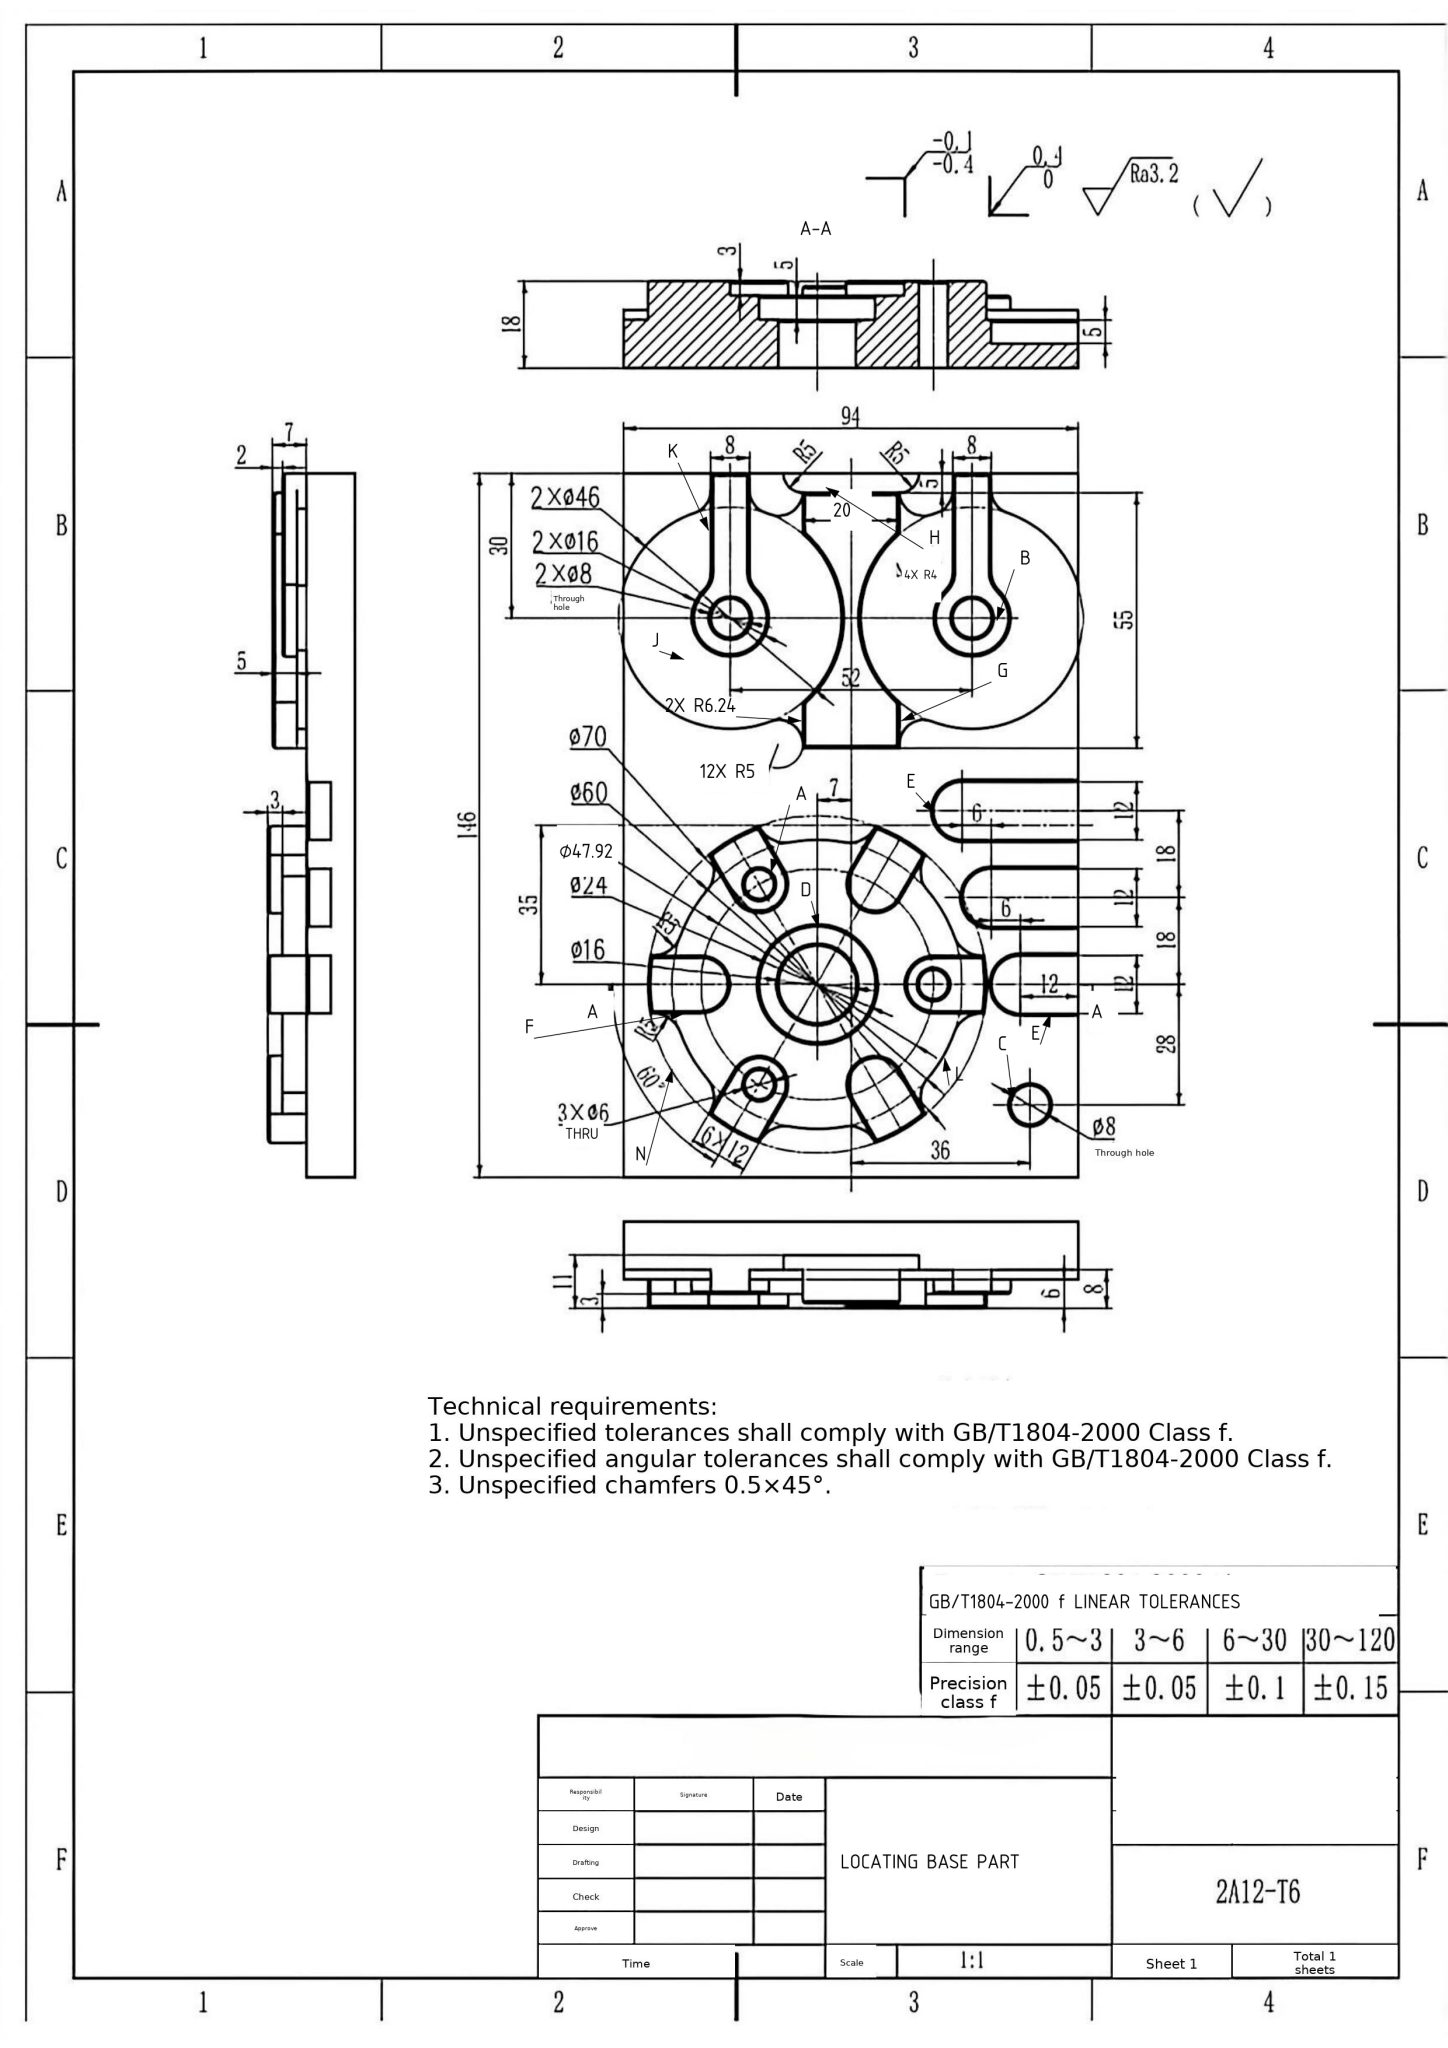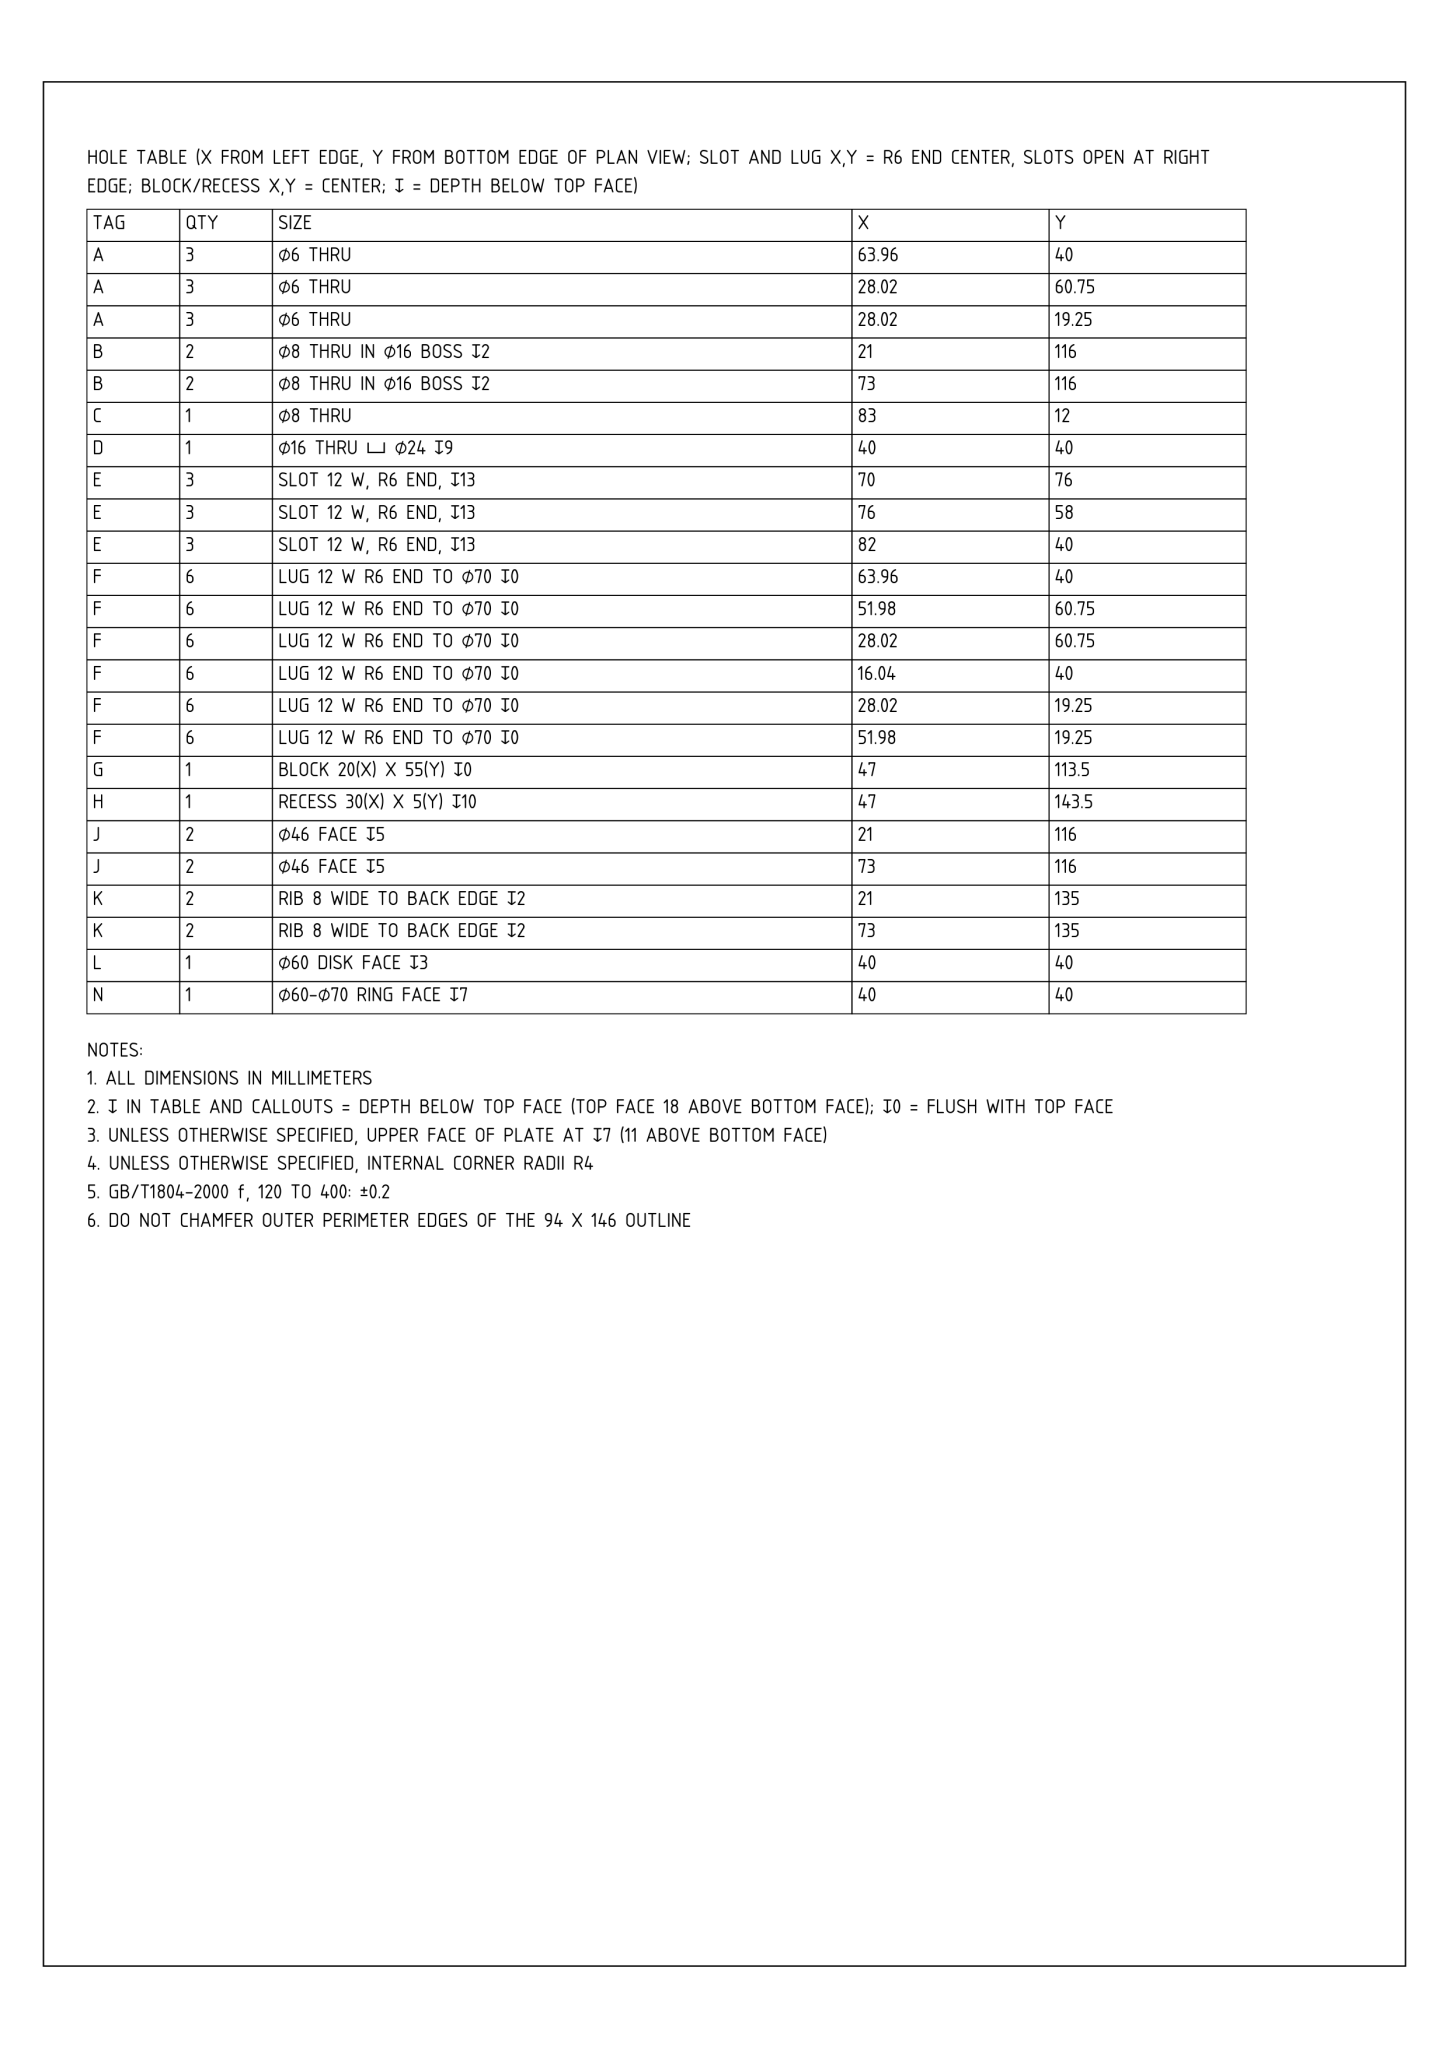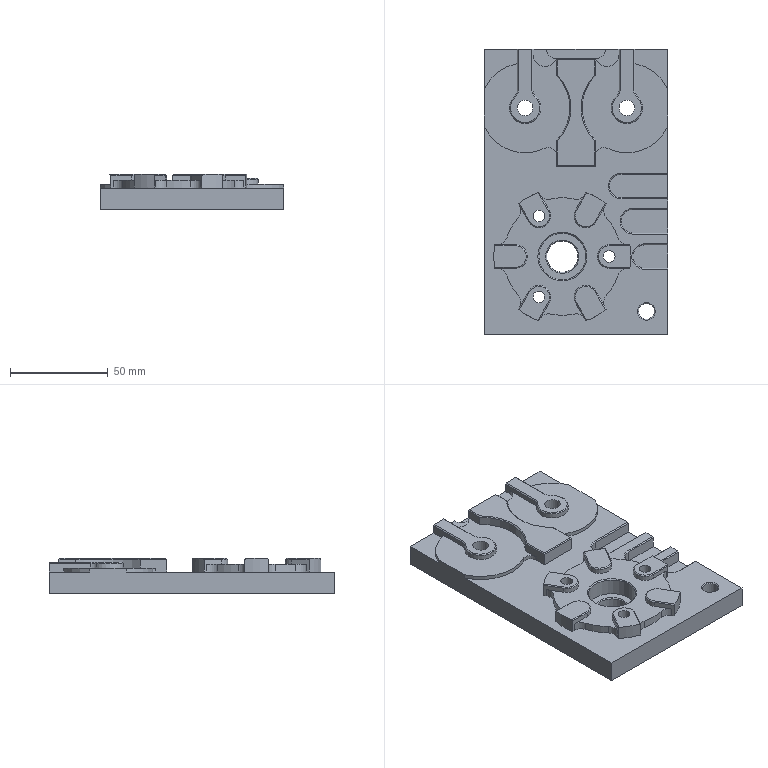Part | NX | mm | 1 solid | 162 faces | box 94 x 146 x 18 mm | volume 167485 mm3 | plane 83 | cylinder 59 | cone 20 | commonest cylinder face diameters 10 x14 12 x9 8 x9 46 x6 70 x6 60 x6 16 x3 6 x3